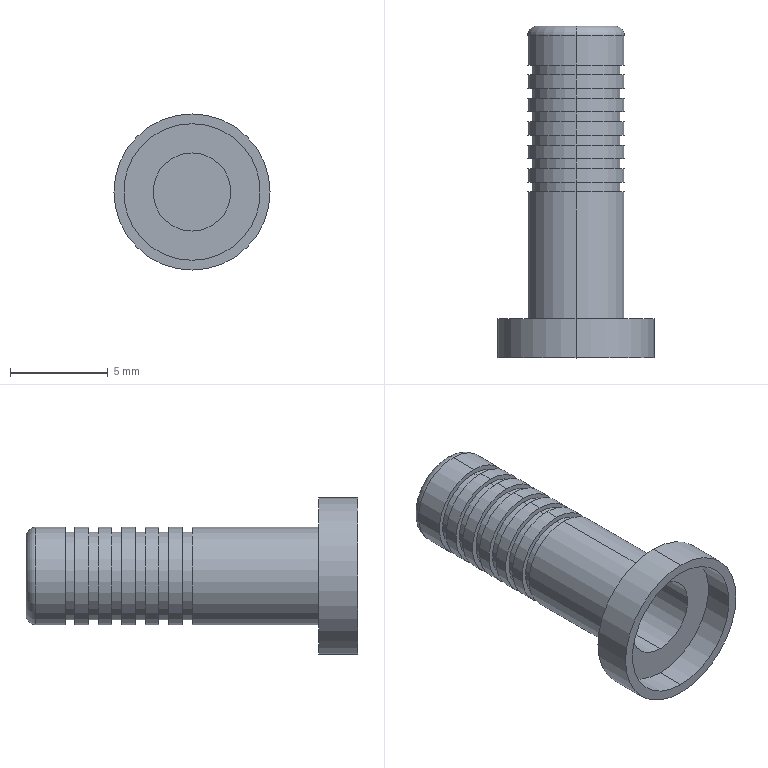Component | SolidWorks | PenTailCap-1 | 1 solid | 51 faces | volume 137 mm3 | cylinder 32 | plane 17 | torus 2 | commonest cylinder face diameters 5 x14 4.5 x12 4 x2 7 x2 8 x2